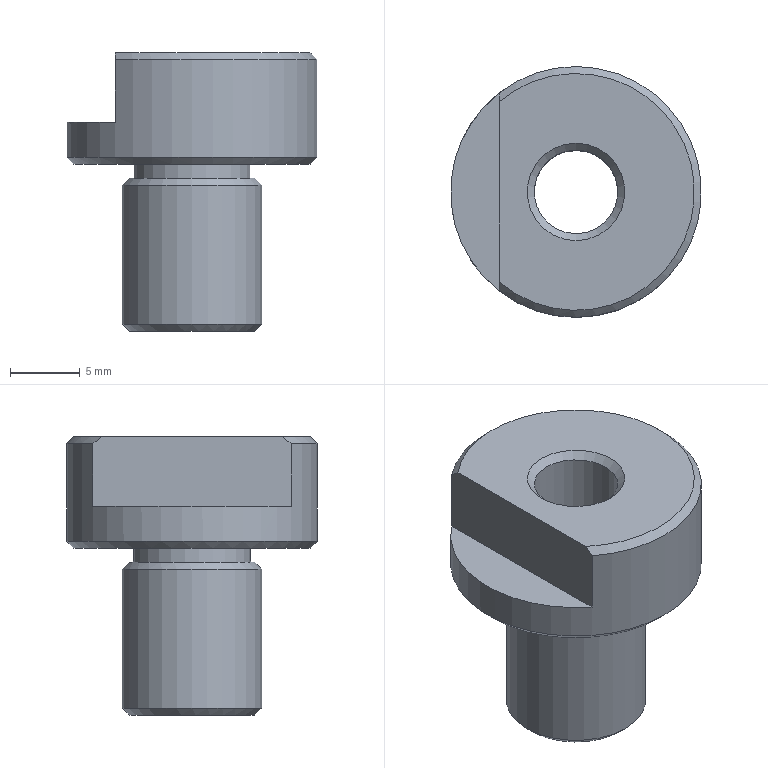Component | NX | DRILL_BUSH | 1 solid | 16 faces | box 18 x 18 x 20 mm | volume 2191 mm3 | plane 6 | cone 6 | cylinder 4 | commonest cylinder face diameters 18 x1 8.4 x1 10 x1 6 x1
STEP:
#1=CARTESIAN_POINT('',(0.,0.,0.));
#2=DIRECTION('',(0.,0.,1.));
#3=DIRECTION('',(1.,0.,0.));
#4=AXIS2_PLACEMENT_3D('',#1,#2,#3);
#5=CARTESIAN_POINT('',(12.,9.,-4.5));
#6=VERTEX_POINT('',#5);
#7=CARTESIAN_POINT('',(6.5,-7.124,-4.5));
#8=VERTEX_POINT('',#7);
#9=CARTESIAN_POINT('',(12.,0.,-4.5));
#10=DIRECTION('',(0.,0.,1.));
#11=DIRECTION('',(0.,1.,0.));
#12=AXIS2_PLACEMENT_3D('',#9,#10,#11);
#13=CIRCLE('',#12,9.);
#14=CARTESIAN_POINT('',(12.,0.,3.));
#15=DIRECTION('',(0.,0.,-1.));
#16=DIRECTION('',(0.,-1.,0.));
#17=AXIS2_PLACEMENT_3D('',#14,#15,#16);
#18=CYLINDRICAL_SURFACE('',#17,9.);
#19=CARTESIAN_POINT('',(3.142,7.5));
#20=DIRECTION('',(-1.,0.));
#21=VECTOR('',#20,1.);
#22=LINE('',#19,#21);
#23=(GEOMETRIC_REPRESENTATION_CONTEXT(2)PARAMETRIC_REPRESENTATION_CONTEXT()REPRESENTATION_CONTEXT('',''));
#24=DEFINITIONAL_REPRESENTATION('',(#22),#23);
#25=PCURVE('',#18,#24);
#26=CARTESIAN_POINT('',(12.,0.,-4.5));
#27=DIRECTION('',(0.,0.,1.));
#28=DIRECTION('',(0.,1.,0.));
#29=AXIS2_PLACEMENT_3D('',#26,#27,#28);
#30=CONICAL_SURFACE('',#29,9.,0.7854);
#31=CARTESIAN_POINT('',(0.,0.));
#32=DIRECTION('',(1.,0.));
#33=VECTOR('',#32,1.);
#34=LINE('',#31,#33);
#35=(GEOMETRIC_REPRESENTATION_CONTEXT(2)PARAMETRIC_REPRESENTATION_CONTEXT()REPRESENTATION_CONTEXT('',''));
#36=DEFINITIONAL_REPRESENTATION('',(#34),#35);
#37=PCURVE('',#30,#36);
#38=SURFACE_CURVE('',#13,(#25,#37),.PCURVE_S1.);
#39=EDGE_CURVE('',#6,#8,#38,.T.);
#40=ORIENTED_EDGE('',*,*,#39,.T.);
#41=CARTESIAN_POINT('',(6.5,-7.124,-2.));
#42=VERTEX_POINT('',#41);
#43=CARTESIAN_POINT('',(6.5,-7.124,-2.));
#44=CARTESIAN_POINT('',(6.5,-7.124,-4.5));
#45=B_SPLINE_CURVE_WITH_KNOTS('',1,(#43,#44),.UNSPECIFIED.,.F.,.F.,(2,2),(5.,7.5),.PIECEWISE_BEZIER_KNOTS.);
#46=CARTESIAN_POINT('',(0.6575,0.));
#47=DIRECTION('',(0.,1.));
#48=VECTOR('',#47,1.);
#49=LINE('',#46,#48);
#50=(GEOMETRIC_REPRESENTATION_CONTEXT(2)PARAMETRIC_REPRESENTATION_CONTEXT()REPRESENTATION_CONTEXT('',''));
#51=DEFINITIONAL_REPRESENTATION('',(#49),#50);
#52=PCURVE('',#18,#51);
#53=CARTESIAN_POINT('',(6.941,0.));
#54=DIRECTION('',(0.,1.));
#55=VECTOR('',#54,1.);
#56=LINE('',#53,#55);
#57=(GEOMETRIC_REPRESENTATION_CONTEXT(2)PARAMETRIC_REPRESENTATION_CONTEXT()REPRESENTATION_CONTEXT('',''));
#58=DEFINITIONAL_REPRESENTATION('',(#56),#57);
#59=PCURVE('',#18,#58);
#60=SEAM_CURVE('',#45,(#52,#59),.PCURVE_S1.);
#61=EDGE_CURVE('',#42,#8,#60,.T.);
#62=ORIENTED_EDGE('',*,*,#61,.F.);
#63=CARTESIAN_POINT('',(6.5,7.124,-2.));
#64=VERTEX_POINT('',#63);
#65=CARTESIAN_POINT('',(12.,0.,-2.));
#66=DIRECTION('',(0.,0.,1.));
#67=DIRECTION('',(0.,1.,0.));
#68=AXIS2_PLACEMENT_3D('',#65,#66,#67);
#69=CIRCLE('',#68,9.);
#70=CARTESIAN_POINT('',(3.142,5.));
#71=DIRECTION('',(-1.,0.));
#72=VECTOR('',#71,1.);
#73=LINE('',#70,#72);
#74=(GEOMETRIC_REPRESENTATION_CONTEXT(2)PARAMETRIC_REPRESENTATION_CONTEXT()REPRESENTATION_CONTEXT('',''));
#75=DEFINITIONAL_REPRESENTATION('',(#73),#74);
#76=PCURVE('',#18,#75);
#77=CARTESIAN_POINT('',(12.,0.,-2.));
#78=DIRECTION('',(0.,0.,1.));
#79=DIRECTION('',(0.,1.,0.));
#80=AXIS2_PLACEMENT_3D('',#77,#78,#79);
#81=PLANE('',#80);
#82=CARTESIAN_POINT('',(0.,0.));
#83=DIRECTION('',(1.,0.));
#84=AXIS2_PLACEMENT_2D('',#82,#83);
#85=CIRCLE('',#84,9.);
#86=(GEOMETRIC_REPRESENTATION_CONTEXT(2)PARAMETRIC_REPRESENTATION_CONTEXT()REPRESENTATION_CONTEXT('',''));
#87=DEFINITIONAL_REPRESENTATION('',(#85),#86);
#88=PCURVE('',#81,#87);
#89=SURFACE_CURVE('',#69,(#76,#88),.PCURVE_S1.);
#90=EDGE_CURVE('',#64,#42,#89,.T.);
#91=ORIENTED_EDGE('',*,*,#90,.F.);
#92=CARTESIAN_POINT('',(6.5,7.124,2.5));
#93=VERTEX_POINT('',#92);
#94=CARTESIAN_POINT('',(6.5,7.124,3.));
#95=DIRECTION('',(0.,0.,1.));
#96=VECTOR('',#95,1.);
#97=LINE('',#94,#96);
#98=CARTESIAN_POINT('',(2.484,0.));
#99=DIRECTION('',(0.,-1.));
#100=VECTOR('',#99,1.);
#101=LINE('',#98,#100);
#102=(GEOMETRIC_REPRESENTATION_CONTEXT(2)PARAMETRIC_REPRESENTATION_CONTEXT()REPRESENTATION_CONTEXT('',''));
#103=DEFINITIONAL_REPRESENTATION('',(#101),#102);
#104=PCURVE('',#18,#103);
#105=CARTESIAN_POINT('',(6.5,-9.7,-2.));
#106=DIRECTION('',(1.,0.,0.));
#107=DIRECTION('',(-0.,1.,0.));
#108=AXIS2_PLACEMENT_3D('',#105,#106,#107);
#109=PLANE('',#108);
#110=CARTESIAN_POINT('',(16.824,5.));
#111=DIRECTION('',(0.,1.));
#112=VECTOR('',#111,1.);
#113=LINE('',#110,#112);
#114=(GEOMETRIC_REPRESENTATION_CONTEXT(2)PARAMETRIC_REPRESENTATION_CONTEXT()REPRESENTATION_CONTEXT('',''));
#115=DEFINITIONAL_REPRESENTATION('',(#113),#114);
#116=PCURVE('',#109,#115);
#117=SURFACE_CURVE('',#97,(#104,#116),.PCURVE_S1.);
#118=EDGE_CURVE('',#64,#93,#117,.T.);
#119=ORIENTED_EDGE('',*,*,#118,.T.);
#120=CARTESIAN_POINT('',(6.5,-7.124,2.5));
#121=VERTEX_POINT('',#120);
#122=CARTESIAN_POINT('',(12.,0.,2.5));
#123=DIRECTION('',(0.,0.,-1.));
#124=DIRECTION('',(0.,1.,0.));
#125=AXIS2_PLACEMENT_3D('',#122,#123,#124);
#126=CIRCLE('',#125,9.);
#127=CARTESIAN_POINT('',(-3.142,0.5));
#128=DIRECTION('',(1.,0.));
#129=VECTOR('',#128,1.);
#130=LINE('',#127,#129);
#131=(GEOMETRIC_REPRESENTATION_CONTEXT(2)PARAMETRIC_REPRESENTATION_CONTEXT()REPRESENTATION_CONTEXT('',''));
#132=DEFINITIONAL_REPRESENTATION('',(#130),#131);
#133=PCURVE('',#18,#132);
#134=CARTESIAN_POINT('',(12.,0.,3.));
#135=DIRECTION('',(0.,0.,-1.));
#136=DIRECTION('',(0.,-1.,0.));
#137=AXIS2_PLACEMENT_3D('',#134,#135,#136);
#138=CONICAL_SURFACE('',#137,8.5,0.7854);
#139=CARTESIAN_POINT('',(-3.142,0.5));
#140=DIRECTION('',(1.,0.));
#141=VECTOR('',#140,1.);
#142=LINE('',#139,#141);
#143=(GEOMETRIC_REPRESENTATION_CONTEXT(2)PARAMETRIC_REPRESENTATION_CONTEXT()REPRESENTATION_CONTEXT('',''));
#144=DEFINITIONAL_REPRESENTATION('',(#142),#143);
#145=PCURVE('',#138,#144);
#146=SURFACE_CURVE('',#126,(#133,#145),.PCURVE_S1.);
#147=EDGE_CURVE('',#93,#121,#146,.T.);
#148=ORIENTED_EDGE('',*,*,#147,.T.);
#149=CARTESIAN_POINT('',(6.5,-7.124,3.));
#150=DIRECTION('',(0.,0.,-1.));
#151=VECTOR('',#150,1.);
#152=LINE('',#149,#151);
#153=CARTESIAN_POINT('',(6.941,0.));
#154=DIRECTION('',(0.,1.));
#155=VECTOR('',#154,1.);
#156=LINE('',#153,#155);
#157=(GEOMETRIC_REPRESENTATION_CONTEXT(2)PARAMETRIC_REPRESENTATION_CONTEXT()REPRESENTATION_CONTEXT('',''));
#158=DEFINITIONAL_REPRESENTATION('',(#156),#157);
#159=PCURVE('',#18,#158);
#160=CARTESIAN_POINT('',(2.576,5.));
#161=DIRECTION('',(0.,-1.));
#162=VECTOR('',#161,1.);
#163=LINE('',#160,#162);
#164=(GEOMETRIC_REPRESENTATION_CONTEXT(2)PARAMETRIC_REPRESENTATION_CONTEXT()REPRESENTATION_CONTEXT('',''));
#165=DEFINITIONAL_REPRESENTATION('',(#163),#164);
#166=PCURVE('',#109,#165);
#167=SURFACE_CURVE('',#152,(#159,#166),.PCURVE_S1.);
#168=EDGE_CURVE('',#121,#42,#167,.T.);
#169=ORIENTED_EDGE('',*,*,#168,.T.);
#170=ORIENTED_EDGE('',*,*,#61,.T.);
#171=CARTESIAN_POINT('',(12.,0.,-4.5));
#172=DIRECTION('',(0.,0.,1.));
#173=DIRECTION('',(0.,1.,0.));
#174=AXIS2_PLACEMENT_3D('',#171,#172,#173);
#175=CIRCLE('',#174,9.);
#176=CARTESIAN_POINT('',(9.425,7.5));
#177=DIRECTION('',(-1.,0.));
#178=VECTOR('',#177,1.);
#179=LINE('',#176,#178);
#180=(GEOMETRIC_REPRESENTATION_CONTEXT(2)PARAMETRIC_REPRESENTATION_CONTEXT()REPRESENTATION_CONTEXT('',''));
#181=DEFINITIONAL_REPRESENTATION('',(#179),#180);
#182=PCURVE('',#18,#181);
#183=CARTESIAN_POINT('',(0.,0.));
#184=DIRECTION('',(1.,0.));
#185=VECTOR('',#184,1.);
#186=LINE('',#183,#185);
#187=(GEOMETRIC_REPRESENTATION_CONTEXT(2)PARAMETRIC_REPRESENTATION_CONTEXT()REPRESENTATION_CONTEXT('',''));
#188=DEFINITIONAL_REPRESENTATION('',(#186),#187);
#189=PCURVE('',#30,#188);
#190=SURFACE_CURVE('',#175,(#182,#189),.PCURVE_S1.);
#191=EDGE_CURVE('',#8,#6,#190,.T.);
#192=ORIENTED_EDGE('',*,*,#191,.T.);
#193=EDGE_LOOP('',(#40,#62,#91,#119,#148,#169,#170,#192));
#194=FACE_BOUND('',#193,.T.);
#195=ADVANCED_FACE('',(#194),#18,.T.);
#196=CARTESIAN_POINT('',(12.,3.5,3.));
#197=VERTEX_POINT('',#196);
#198=CARTESIAN_POINT('',(12.,0.,3.));
#199=DIRECTION('',(0.,0.,-1.));
#200=DIRECTION('',(0.,1.,0.));
#201=AXIS2_PLACEMENT_3D('',#198,#199,#200);
#202=CIRCLE('',#201,3.5);
#203=CARTESIAN_POINT('',(12.,0.,3.));
#204=DIRECTION('',(0.,0.,1.));
#205=DIRECTION('',(0.,1.,0.));
#206=AXIS2_PLACEMENT_3D('',#203,#204,#205);
#207=PLANE('',#206);
#208=CARTESIAN_POINT('',(3.5,0.));
#209=CARTESIAN_POINT('',(3.5,-6.062));
#210=CARTESIAN_POINT('',(-1.75,-3.031));
#211=CARTESIAN_POINT('',(-7.,-0.));
#212=CARTESIAN_POINT('',(-1.75,3.031));
#213=CARTESIAN_POINT('',(3.5,6.062));
#214=CARTESIAN_POINT('',(3.5,0.));
#215=(BOUNDED_CURVE()B_SPLINE_CURVE(2,(#208,#209,#210,#211,#212,#213,#214),.UNSPECIFIED.,.T.,.F.)B_SPLINE_CURVE_WITH_KNOTS((1,2,2,2,2,1),(-2.094,0.,2.094,4.189,6.283,8.378),.UNSPECIFIED.)CURVE()GEOMETRIC_REPRESENTATION_ITEM()RATIONAL_B_SPLINE_CURVE((1.,0.5,1.,0.5,1.,0.5,1.))REPRESENTATION_ITEM(''));
#216=(GEOMETRIC_REPRESENTATION_CONTEXT(2)PARAMETRIC_REPRESENTATION_CONTEXT()REPRESENTATION_CONTEXT('',''));
#217=DEFINITIONAL_REPRESENTATION('',(#215),#216);
#218=PCURVE('',#207,#217);
#219=CARTESIAN_POINT('',(12.,0.,3.));
#220=DIRECTION('',(0.,0.,1.));
#221=DIRECTION('',(0.,1.,0.));
#222=AXIS2_PLACEMENT_3D('',#219,#220,#221);
#223=CONICAL_SURFACE('',#222,3.5,0.7854);
#224=CARTESIAN_POINT('',(6.283,0.));
#225=DIRECTION('',(-1.,0.));
#226=VECTOR('',#225,1.);
#227=LINE('',#224,#226);
#228=(GEOMETRIC_REPRESENTATION_CONTEXT(2)PARAMETRIC_REPRESENTATION_CONTEXT()REPRESENTATION_CONTEXT('',''));
#229=DEFINITIONAL_REPRESENTATION('',(#227),#228);
#230=PCURVE('',#223,#229);
#231=SURFACE_CURVE('',#202,(#218,#230),.PCURVE_S1.);
#232=EDGE_CURVE('',#197,#197,#231,.T.);
#233=ORIENTED_EDGE('',*,*,#232,.T.);
#234=EDGE_LOOP('',(#233));
#235=FACE_BOUND('',#234,.T.);
#236=CARTESIAN_POINT('',(6.5,-6.481,3.));
#237=VERTEX_POINT('',#236);
#238=CARTESIAN_POINT('',(6.5,6.481,3.));
#239=VERTEX_POINT('',#238);
#240=CARTESIAN_POINT('',(6.5,-9.7,3.));
#241=DIRECTION('',(-0.,1.,0.));
#242=VECTOR('',#241,1.);
#243=LINE('',#240,#242);
#244=CARTESIAN_POINT('',(-9.7,5.5));
#245=DIRECTION('',(1.,0.));
#246=VECTOR('',#245,1.);
#247=LINE('',#244,#246);
#248=(GEOMETRIC_REPRESENTATION_CONTEXT(2)PARAMETRIC_REPRESENTATION_CONTEXT()REPRESENTATION_CONTEXT('',''));
#249=DEFINITIONAL_REPRESENTATION('',(#247),#248);
#250=PCURVE('',#207,#249);
#251=CARTESIAN_POINT('',(0.,5.));
#252=DIRECTION('',(1.,0.));
#253=VECTOR('',#252,1.);
#254=LINE('',#251,#253);
#255=(GEOMETRIC_REPRESENTATION_CONTEXT(2)PARAMETRIC_REPRESENTATION_CONTEXT()REPRESENTATION_CONTEXT('',''));
#256=DEFINITIONAL_REPRESENTATION('',(#254),#255);
#257=PCURVE('',#109,#256);
#258=SURFACE_CURVE('',#243,(#250,#257),.PCURVE_S1.);
#259=EDGE_CURVE('',#237,#239,#258,.T.);
#260=ORIENTED_EDGE('',*,*,#259,.F.);
#261=CARTESIAN_POINT('',(12.,0.,3.));
#262=DIRECTION('',(0.,0.,1.));
#263=DIRECTION('',(0.,1.,0.));
#264=AXIS2_PLACEMENT_3D('',#261,#262,#263);
#265=CIRCLE('',#264,8.5);
#266=CARTESIAN_POINT('',(0.,0.));
#267=DIRECTION('',(1.,0.));
#268=AXIS2_PLACEMENT_2D('',#266,#267);
#269=CIRCLE('',#268,8.5);
#270=(GEOMETRIC_REPRESENTATION_CONTEXT(2)PARAMETRIC_REPRESENTATION_CONTEXT()REPRESENTATION_CONTEXT('',''));
#271=DEFINITIONAL_REPRESENTATION('',(#269),#270);
#272=PCURVE('',#207,#271);
#273=CARTESIAN_POINT('',(9.425,0.));
#274=DIRECTION('',(-1.,0.));
#275=VECTOR('',#274,1.);
#276=LINE('',#273,#275);
#277=(GEOMETRIC_REPRESENTATION_CONTEXT(2)PARAMETRIC_REPRESENTATION_CONTEXT()REPRESENTATION_CONTEXT('',''));
#278=DEFINITIONAL_REPRESENTATION('',(#276),#277);
#279=PCURVE('',#138,#278);
#280=SURFACE_CURVE('',#265,(#272,#279),.PCURVE_S1.);
#281=EDGE_CURVE('',#237,#239,#280,.T.);
#282=ORIENTED_EDGE('',*,*,#281,.T.);
#283=EDGE_LOOP('',(#260,#282));
#284=FACE_BOUND('',#283,.T.);
#285=ADVANCED_FACE('',(#235,#284),#207,.T.);
#286=CARTESIAN_POINT('',(12.,8.5,-5.));
#287=VERTEX_POINT('',#286);
#288=CARTESIAN_POINT('',(12.,0.,-5.));
#289=DIRECTION('',(0.,0.,-1.));
#290=DIRECTION('',(0.,1.,0.));
#291=AXIS2_PLACEMENT_3D('',#288,#289,#290);
#292=CIRCLE('',#291,8.5);
#293=CARTESIAN_POINT('',(12.,0.,-5.));
#294=DIRECTION('',(0.,0.,1.));
#295=DIRECTION('',(0.,1.,0.));
#296=AXIS2_PLACEMENT_3D('',#293,#294,#295);
#297=PLANE('',#296);
#298=CARTESIAN_POINT('',(8.5,0.));
#299=CARTESIAN_POINT('',(8.5,-14.722));
#300=CARTESIAN_POINT('',(-4.25,-7.361));
#301=CARTESIAN_POINT('',(-17.,-0.));
#302=CARTESIAN_POINT('',(-4.25,7.361));
#303=CARTESIAN_POINT('',(8.5,14.722));
#304=CARTESIAN_POINT('',(8.5,0.));
#305=(BOUNDED_CURVE()B_SPLINE_CURVE(2,(#298,#299,#300,#301,#302,#303,#304),.UNSPECIFIED.,.T.,.F.)B_SPLINE_CURVE_WITH_KNOTS((1,2,2,2,2,1),(-2.094,0.,2.094,4.189,6.283,8.378),.UNSPECIFIED.)CURVE()GEOMETRIC_REPRESENTATION_ITEM()RATIONAL_B_SPLINE_CURVE((1.,0.5,1.,0.5,1.,0.5,1.))REPRESENTATION_ITEM(''));
#306=(GEOMETRIC_REPRESENTATION_CONTEXT(2)PARAMETRIC_REPRESENTATION_CONTEXT()REPRESENTATION_CONTEXT('',''));
#307=DEFINITIONAL_REPRESENTATION('',(#305),#306);
#308=PCURVE('',#297,#307);
#309=CARTESIAN_POINT('',(6.283,-0.5));
#310=DIRECTION('',(-1.,0.));
#311=VECTOR('',#310,1.);
#312=LINE('',#309,#311);
#313=(GEOMETRIC_REPRESENTATION_CONTEXT(2)PARAMETRIC_REPRESENTATION_CONTEXT()REPRESENTATION_CONTEXT('',''));
#314=DEFINITIONAL_REPRESENTATION('',(#312),#313);
#315=PCURVE('',#30,#314);
#316=SURFACE_CURVE('',#292,(#308,#315),.PCURVE_S1.);
#317=EDGE_CURVE('',#287,#287,#316,.T.);
#318=ORIENTED_EDGE('',*,*,#317,.T.);
#319=EDGE_LOOP('',(#318));
#320=FACE_BOUND('',#319,.T.);
#321=CARTESIAN_POINT('',(12.,-4.2,-5.));
#322=VERTEX_POINT('',#321);
#323=CARTESIAN_POINT('',(12.,0.,-5.));
#324=DIRECTION('',(0.,0.,-1.));
#325=DIRECTION('',(0.,-1.,0.));
#326=AXIS2_PLACEMENT_3D('',#323,#324,#325);
#327=CIRCLE('',#326,4.2);
#328=CARTESIAN_POINT('',(-4.2,0.));
#329=CARTESIAN_POINT('',(-4.2,7.275));
#330=CARTESIAN_POINT('',(2.1,3.637));
#331=CARTESIAN_POINT('',(8.4,0.));
#332=CARTESIAN_POINT('',(2.1,-3.637));
#333=CARTESIAN_POINT('',(-4.2,-7.275));
#334=CARTESIAN_POINT('',(-4.2,0.));
#335=(BOUNDED_CURVE()B_SPLINE_CURVE(2,(#328,#329,#330,#331,#332,#333,#334),.UNSPECIFIED.,.T.,.F.)B_SPLINE_CURVE_WITH_KNOTS((1,2,2,2,2,1),(-2.094,0.,2.094,4.189,6.283,8.378),.UNSPECIFIED.)CURVE()GEOMETRIC_REPRESENTATION_ITEM()RATIONAL_B_SPLINE_CURVE((1.,0.5,1.,0.5,1.,0.5,1.))REPRESENTATION_ITEM(''));
#336=(GEOMETRIC_REPRESENTATION_CONTEXT(2)PARAMETRIC_REPRESENTATION_CONTEXT()REPRESENTATION_CONTEXT('',''));
#337=DEFINITIONAL_REPRESENTATION('',(#335),#336);
#338=PCURVE('',#297,#337);
#339=CARTESIAN_POINT('',(12.,0.,-5.5));
#340=DIRECTION('',(0.,0.,-1.));
#341=DIRECTION('',(0.,-1.,0.));
#342=AXIS2_PLACEMENT_3D('',#339,#340,#341);
#343=CYLINDRICAL_SURFACE('',#342,4.2);
#344=CARTESIAN_POINT('',(0.,-0.5));
#345=DIRECTION('',(1.,0.));
#346=VECTOR('',#345,1.);
#347=LINE('',#344,#346);
#348=(GEOMETRIC_REPRESENTATION_CONTEXT(2)PARAMETRIC_REPRESENTATION_CONTEXT()REPRESENTATION_CONTEXT('',''));
#349=DEFINITIONAL_REPRESENTATION('',(#347),#348);
#350=PCURVE('',#343,#349);
#351=SURFACE_CURVE('',#327,(#338,#350),.PCURVE_S1.);
#352=EDGE_CURVE('',#322,#322,#351,.T.);
#353=ORIENTED_EDGE('',*,*,#352,.F.);
#354=EDGE_LOOP('',(#353));
#355=FACE_BOUND('',#354,.T.);
#356=ADVANCED_FACE('',(#320,#355),#297,.F.);
#357=ORIENTED_EDGE('',*,*,#90,.T.);
#358=CARTESIAN_POINT('',(6.5,-9.7,-2.));
#359=DIRECTION('',(0.,-1.,0.));
#360=VECTOR('',#359,1.);
#361=LINE('',#358,#360);
#362=CARTESIAN_POINT('',(-9.7,5.5));
#363=DIRECTION('',(-1.,-0.));
#364=VECTOR('',#363,1.);
#365=LINE('',#362,#364);
#366=(GEOMETRIC_REPRESENTATION_CONTEXT(2)PARAMETRIC_REPRESENTATION_CONTEXT()REPRESENTATION_CONTEXT('',''));
#367=DEFINITIONAL_REPRESENTATION('',(#365),#366);
#368=PCURVE('',#81,#367);
#369=CARTESIAN_POINT('',(0.,0.));
#370=DIRECTION('',(-1.,0.));
#371=VECTOR('',#370,1.);
#372=LINE('',#369,#371);
#373=(GEOMETRIC_REPRESENTATION_CONTEXT(2)PARAMETRIC_REPRESENTATION_CONTEXT()REPRESENTATION_CONTEXT('',''));
#374=DEFINITIONAL_REPRESENTATION('',(#372),#373);
#375=PCURVE('',#109,#374);
#376=SURFACE_CURVE('',#361,(#368,#375),.PCURVE_S1.);
#377=EDGE_CURVE('',#64,#42,#376,.T.);
#378=ORIENTED_EDGE('',*,*,#377,.F.);
#379=EDGE_LOOP('',(#357,#378));
#380=FACE_BOUND('',#379,.T.);
#381=ADVANCED_FACE('',(#380),#81,.T.);
#382=ORIENTED_EDGE('',*,*,#259,.T.);
#383=CARTESIAN_POINT('',(6.5,6.481,3.));
#384=CARTESIAN_POINT('',(6.5,6.697,2.835));
#385=CARTESIAN_POINT('',(6.5,6.911,2.669));
#386=CARTESIAN_POINT('',(6.5,7.124,2.5));
#387=B_SPLINE_CURVE_WITH_KNOTS('',3,(#383,#384,#385,#386),.UNSPECIFIED.,.F.,.F.,(4,4),(0.,1.),.PIECEWISE_BEZIER_KNOTS.);
#388=CARTESIAN_POINT('',(16.181,5.));
#389=CARTESIAN_POINT('',(16.397,4.835));
#390=CARTESIAN_POINT('',(16.611,4.669));
#391=CARTESIAN_POINT('',(16.824,4.5));
#392=B_SPLINE_CURVE_WITH_KNOTS('',3,(#388,#389,#390,#391),.UNSPECIFIED.,.F.,.F.,(4,4),(0.,1.),.PIECEWISE_BEZIER_KNOTS.);
#393=(GEOMETRIC_REPRESENTATION_CONTEXT(2)PARAMETRIC_REPRESENTATION_CONTEXT()REPRESENTATION_CONTEXT('',''));
#394=DEFINITIONAL_REPRESENTATION('',(#392),#393);
#395=PCURVE('',#109,#394);
#396=CARTESIAN_POINT('',(2.438,-0.));
#397=CARTESIAN_POINT('',(2.484,0.5));
#398=B_SPLINE_CURVE_WITH_KNOTS('',1,(#396,#397),.UNSPECIFIED.,.F.,.F.,(2,2),(0.,1.),.PIECEWISE_BEZIER_KNOTS.);
#399=(GEOMETRIC_REPRESENTATION_CONTEXT(2)PARAMETRIC_REPRESENTATION_CONTEXT()REPRESENTATION_CONTEXT('',''));
#400=DEFINITIONAL_REPRESENTATION('',(#398),#399);
#401=PCURVE('',#138,#400);
#402=SURFACE_CURVE('',#387,(#395,#401),.PCURVE_S1.);
#403=EDGE_CURVE('',#239,#93,#402,.T.);
#404=ORIENTED_EDGE('',*,*,#403,.T.);
#405=ORIENTED_EDGE('',*,*,#118,.F.);
#406=ORIENTED_EDGE('',*,*,#377,.T.);
#407=ORIENTED_EDGE('',*,*,#168,.F.);
#408=CARTESIAN_POINT('',(6.5,-7.124,2.5));
#409=CARTESIAN_POINT('',(6.5,-6.911,2.669));
#410=CARTESIAN_POINT('',(6.5,-6.697,2.835));
#411=CARTESIAN_POINT('',(6.5,-6.481,3.));
#412=B_SPLINE_CURVE_WITH_KNOTS('',3,(#408,#409,#410,#411),.UNSPECIFIED.,.F.,.F.,(4,4),(0.,1.),.PIECEWISE_BEZIER_KNOTS.);
#413=CARTESIAN_POINT('',(2.576,4.5));
#414=CARTESIAN_POINT('',(2.789,4.669));
#415=CARTESIAN_POINT('',(3.003,4.835));
#416=CARTESIAN_POINT('',(3.219,5.));
#417=B_SPLINE_CURVE_WITH_KNOTS('',3,(#413,#414,#415,#416),.UNSPECIFIED.,.F.,.F.,(4,4),(0.,1.),.PIECEWISE_BEZIER_KNOTS.);
#418=(GEOMETRIC_REPRESENTATION_CONTEXT(2)PARAMETRIC_REPRESENTATION_CONTEXT()REPRESENTATION_CONTEXT('',''));
#419=DEFINITIONAL_REPRESENTATION('',(#417),#418);
#420=PCURVE('',#109,#419);
#421=CARTESIAN_POINT('',(6.941,0.5));
#422=CARTESIAN_POINT('',(6.987,-0.));
#423=B_SPLINE_CURVE_WITH_KNOTS('',1,(#421,#422),.UNSPECIFIED.,.F.,.F.,(2,2),(0.,1.),.PIECEWISE_BEZIER_KNOTS.);
#424=(GEOMETRIC_REPRESENTATION_CONTEXT(2)PARAMETRIC_REPRESENTATION_CONTEXT()REPRESENTATION_CONTEXT('',''));
#425=DEFINITIONAL_REPRESENTATION('',(#423),#424);
#426=PCURVE('',#138,#425);
#427=SURFACE_CURVE('',#412,(#420,#426),.PCURVE_S1.);
#428=EDGE_CURVE('',#121,#237,#427,.T.);
#429=ORIENTED_EDGE('',*,*,#428,.T.);
#430=EDGE_LOOP('',(#382,#404,#405,#406,#407,#429));
#431=FACE_BOUND('',#430,.T.);
#432=ADVANCED_FACE('',(#431),#109,.F.);
#433=CARTESIAN_POINT('',(12.,-4.5,-6.));
#434=VERTEX_POINT('',#433);
#435=CARTESIAN_POINT('',(12.,0.,-6.));
#436=DIRECTION('',(0.,0.,1.));
#437=DIRECTION('',(0.,-1.,0.));
#438=AXIS2_PLACEMENT_3D('',#435,#436,#437);
#439=CIRCLE('',#438,4.5);
#440=CARTESIAN_POINT('',(12.,0.,-6.));
#441=DIRECTION('',(0.,0.,-1.));
#442=DIRECTION('',(0.,-1.,0.));
#443=AXIS2_PLACEMENT_3D('',#440,#441,#442);
#444=PLANE('',#443);
#445=CARTESIAN_POINT('',(4.5,0.));
#446=CARTESIAN_POINT('',(4.5,-7.794));
#447=CARTESIAN_POINT('',(-2.25,-3.897));
#448=CARTESIAN_POINT('',(-9.,-0.));
#449=CARTESIAN_POINT('',(-2.25,3.897));
#450=CARTESIAN_POINT('',(4.5,7.794));
#451=CARTESIAN_POINT('',(4.5,0.));
#452=(BOUNDED_CURVE()B_SPLINE_CURVE(2,(#445,#446,#447,#448,#449,#450,#451),.UNSPECIFIED.,.T.,.F.)B_SPLINE_CURVE_WITH_KNOTS((1,2,2,2,2,1),(-2.094,0.,2.094,4.189,6.283,8.378),.UNSPECIFIED.)CURVE()GEOMETRIC_REPRESENTATION_ITEM()RATIONAL_B_SPLINE_CURVE((1.,0.5,1.,0.5,1.,0.5,1.))REPRESENTATION_ITEM(''));
#453=(GEOMETRIC_REPRESENTATION_CONTEXT(2)PARAMETRIC_REPRESENTATION_CONTEXT()REPRESENTATION_CONTEXT('',''));
#454=DEFINITIONAL_REPRESENTATION('',(#452),#453);
#455=PCURVE('',#444,#454);
#456=CARTESIAN_POINT('',(12.,0.,-6.5));
#457=DIRECTION('',(0.,0.,-1.));
#458=DIRECTION('',(0.,-1.,0.));
#459=AXIS2_PLACEMENT_3D('',#456,#457,#458);
#460=CONICAL_SURFACE('',#459,5.,0.7854);
#461=CARTESIAN_POINT('',(6.283,-0.5));
#462=DIRECTION('',(-1.,0.));
#463=VECTOR('',#462,1.);
#464=LINE('',#461,#463);
#465=(GEOMETRIC_REPRESENTATION_CONTEXT(2)PARAMETRIC_REPRESENTATION_CONTEXT()REPRESENTATION_CONTEXT('',''));
#466=DEFINITIONAL_REPRESENTATION('',(#464),#465);
#467=PCURVE('',#460,#466);
#468=SURFACE_CURVE('',#439,(#455,#467),.PCURVE_S1.);
#469=EDGE_CURVE('',#434,#434,#468,.T.);
#470=ORIENTED_EDGE('',*,*,#469,.T.);
#471=EDGE_LOOP('',(#470));
#472=FACE_BOUND('',#471,.T.);
#473=CARTESIAN_POINT('',(12.,-4.2,-6.));
#474=VERTEX_POINT('',#473);
#475=CARTESIAN_POINT('',(12.,0.,-6.));
#476=DIRECTION('',(0.,0.,1.));
#477=DIRECTION('',(0.,-1.,0.));
#478=AXIS2_PLACEMENT_3D('',#475,#476,#477);
#479=CIRCLE('',#478,4.2);
#480=CARTESIAN_POINT('',(4.2,0.));
#481=CARTESIAN_POINT('',(4.2,-7.275));
#482=CARTESIAN_POINT('',(-2.1,-3.637));
#483=CARTESIAN_POINT('',(-8.4,-0.));
#484=CARTESIAN_POINT('',(-2.1,3.637));
#485=CARTESIAN_POINT('',(4.2,7.275));
#486=CARTESIAN_POINT('',(4.2,0.));
#487=(BOUNDED_CURVE()B_SPLINE_CURVE(2,(#480,#481,#482,#483,#484,#485,#486),.UNSPECIFIED.,.T.,.F.)B_SPLINE_CURVE_WITH_KNOTS((1,2,2,2,2,1),(-2.094,0.,2.094,4.189,6.283,8.378),.UNSPECIFIED.)CURVE()GEOMETRIC_REPRESENTATION_ITEM()RATIONAL_B_SPLINE_CURVE((1.,0.5,1.,0.5,1.,0.5,1.))REPRESENTATION_ITEM(''));
#488=(GEOMETRIC_REPRESENTATION_CONTEXT(2)PARAMETRIC_REPRESENTATION_CONTEXT()REPRESENTATION_CONTEXT('',''));
#489=DEFINITIONAL_REPRESENTATION('',(#487),#488);
#490=PCURVE('',#444,#489);
#491=CARTESIAN_POINT('',(6.283,0.5));
#492=DIRECTION('',(-1.,0.));
#493=VECTOR('',#492,1.);
#494=LINE('',#491,#493);
#495=(GEOMETRIC_REPRESENTATION_CONTEXT(2)PARAMETRIC_REPRESENTATION_CONTEXT()REPRESENTATION_CONTEXT('',''));
#496=DEFINITIONAL_REPRESENTATION('',(#494),#495);
#497=PCURVE('',#343,#496);
#498=SURFACE_CURVE('',#479,(#490,#497),.PCURVE_S1.);
#499=EDGE_CURVE('',#474,#474,#498,.T.);
#500=ORIENTED_EDGE('',*,*,#499,.F.);
#501=EDGE_LOOP('',(#500));
#502=FACE_BOUND('',#501,.T.);
#503=ADVANCED_FACE('',(#472,#502),#444,.F.);
#504=ORIENTED_EDGE('',*,*,#499,.T.);
#505=CARTESIAN_POINT('',(12.,-4.2,-5.));
#506=CARTESIAN_POINT('',(12.,-4.2,-6.));
#507=B_SPLINE_CURVE_WITH_KNOTS('',1,(#505,#506),.UNSPECIFIED.,.F.,.F.,(2,2),(-0.5,0.5),.PIECEWISE_BEZIER_KNOTS.);
#508=CARTESIAN_POINT('',(0.,0.));
#509=DIRECTION('',(0.,1.));
#510=VECTOR('',#509,1.);
#511=LINE('',#508,#510);
#512=(GEOMETRIC_REPRESENTATION_CONTEXT(2)PARAMETRIC_REPRESENTATION_CONTEXT()REPRESENTATION_CONTEXT('',''));
#513=DEFINITIONAL_REPRESENTATION('',(#511),#512);
#514=PCURVE('',#343,#513);
#515=CARTESIAN_POINT('',(6.283,0.));
#516=DIRECTION('',(0.,1.));
#517=VECTOR('',#516,1.);
#518=LINE('',#515,#517);
#519=(GEOMETRIC_REPRESENTATION_CONTEXT(2)PARAMETRIC_REPRESENTATION_CONTEXT()REPRESENTATION_CONTEXT('',''));
#520=DEFINITIONAL_REPRESENTATION('',(#518),#519);
#521=PCURVE('',#343,#520);
#522=SEAM_CURVE('',#507,(#514,#521),.PCURVE_S1.);
#523=EDGE_CURVE('',#322,#474,#522,.T.);
#524=ORIENTED_EDGE('',*,*,#523,.F.);
#525=ORIENTED_EDGE('',*,*,#352,.T.);
#526=ORIENTED_EDGE('',*,*,#523,.T.);
#527=EDGE_LOOP('',(#504,#524,#525,#526));
#528=FACE_BOUND('',#527,.T.);
#529=ADVANCED_FACE('',(#528),#343,.T.);
#530=CARTESIAN_POINT('',(12.,3.5,-17.));
#531=VERTEX_POINT('',#530);
#532=CARTESIAN_POINT('',(12.,0.,-17.));
#533=DIRECTION('',(0.,0.,1.));
#534=DIRECTION('',(0.,1.,0.));
#535=AXIS2_PLACEMENT_3D('',#532,#533,#534);
#536=CIRCLE('',#535,3.5);
#537=CARTESIAN_POINT('',(12.,0.,-17.));
#538=DIRECTION('',(0.,0.,1.));
#539=DIRECTION('',(0.,1.,0.));
#540=AXIS2_PLACEMENT_3D('',#537,#538,#539);
#541=PLANE('',#540);
#542=CARTESIAN_POINT('',(0.,0.));
#543=DIRECTION('',(1.,0.));
#544=AXIS2_PLACEMENT_2D('',#542,#543);
#545=CIRCLE('',#544,3.5);
#546=(GEOMETRIC_REPRESENTATION_CONTEXT(2)PARAMETRIC_REPRESENTATION_CONTEXT()REPRESENTATION_CONTEXT('',''));
#547=DEFINITIONAL_REPRESENTATION('',(#545),#546);
#548=PCURVE('',#541,#547);
#549=CARTESIAN_POINT('',(12.,0.,-17.));
#550=DIRECTION('',(0.,0.,-1.));
#551=DIRECTION('',(0.,-1.,0.));
#552=AXIS2_PLACEMENT_3D('',#549,#550,#551);
#553=CONICAL_SURFACE('',#552,3.5,0.7854);
#554=CARTESIAN_POINT('',(9.425,0.));
#555=DIRECTION('',(-1.,0.));
#556=VECTOR('',#555,1.);
#557=LINE('',#554,#556);
#558=(GEOMETRIC_REPRESENTATION_CONTEXT(2)PARAMETRIC_REPRESENTATION_CONTEXT()REPRESENTATION_CONTEXT('',''));
#559=DEFINITIONAL_REPRESENTATION('',(#557),#558);
#560=PCURVE('',#553,#559);
#561=SURFACE_CURVE('',#536,(#548,#560),.PCURVE_S1.);
#562=EDGE_CURVE('',#531,#531,#561,.T.);
#563=ORIENTED_EDGE('',*,*,#562,.T.);
#564=EDGE_LOOP('',(#563));
#565=FACE_BOUND('',#564,.T.);
#566=CARTESIAN_POINT('',(12.,4.5,-17.));
#567=VERTEX_POINT('',#566);
#568=CARTESIAN_POINT('',(12.,0.,-17.));
#569=DIRECTION('',(0.,0.,-1.));
#570=DIRECTION('',(0.,1.,0.));
#571=AXIS2_PLACEMENT_3D('',#568,#569,#570);
#572=CIRCLE('',#571,4.5);
#573=CARTESIAN_POINT('',(4.5,0.));
#574=CARTESIAN_POINT('',(4.5,-7.794));
#575=CARTESIAN_POINT('',(-2.25,-3.897));
#576=CARTESIAN_POINT('',(-9.,-0.));
#577=CARTESIAN_POINT('',(-2.25,3.897));
#578=CARTESIAN_POINT('',(4.5,7.794));
#579=CARTESIAN_POINT('',(4.5,0.));
#580=(BOUNDED_CURVE()B_SPLINE_CURVE(2,(#573,#574,#575,#576,#577,#578,#579),.UNSPECIFIED.,.T.,.F.)B_SPLINE_CURVE_WITH_KNOTS((1,2,2,2,2,1),(-2.094,0.,2.094,4.189,6.283,8.378),.UNSPECIFIED.)CURVE()GEOMETRIC_REPRESENTATION_ITEM()RATIONAL_B_SPLINE_CURVE((1.,0.5,1.,0.5,1.,0.5,1.))REPRESENTATION_ITEM(''));
#581=(GEOMETRIC_REPRESENTATION_CONTEXT(2)PARAMETRIC_REPRESENTATION_CONTEXT()REPRESENTATION_CONTEXT('',''));
#582=DEFINITIONAL_REPRESENTATION('',(#580),#581);
#583=PCURVE('',#541,#582);
#584=CARTESIAN_POINT('',(12.,0.,-16.5));
#585=DIRECTION('',(0.,0.,1.));
#586=DIRECTION('',(0.,1.,0.));
#587=AXIS2_PLACEMENT_3D('',#584,#585,#586);
#588=CONICAL_SURFACE('',#587,5.,0.7854);
#589=CARTESIAN_POINT('',(6.283,-0.5));
#590=DIRECTION('',(-1.,0.));
#591=VECTOR('',#590,1.);
#592=LINE('',#589,#591);
#593=(GEOMETRIC_REPRESENTATION_CONTEXT(2)PARAMETRIC_REPRESENTATION_CONTEXT()REPRESENTATION_CONTEXT('',''));
#594=DEFINITIONAL_REPRESENTATION('',(#592),#593);
#595=PCURVE('',#588,#594);
#596=SURFACE_CURVE('',#572,(#583,#595),.PCURVE_S1.);
#597=EDGE_CURVE('',#567,#567,#596,.T.);
#598=ORIENTED_EDGE('',*,*,#597,.T.);
#599=EDGE_LOOP('',(#598));
#600=FACE_BOUND('',#599,.T.);
#601=ADVANCED_FACE('',(#565,#600),#541,.F.);
#602=CARTESIAN_POINT('',(12.,5.,-16.5));
#603=VERTEX_POINT('',#602);
#604=CARTESIAN_POINT('',(12.,-5.,-16.5));
#605=VERTEX_POINT('',#604);
#606=CARTESIAN_POINT('',(12.,0.,-16.5));
#607=DIRECTION('',(0.,0.,1.));
#608=DIRECTION('',(0.,1.,0.));
#609=AXIS2_PLACEMENT_3D('',#606,#607,#608);
#610=CIRCLE('',#609,5.);
#611=CARTESIAN_POINT('',(12.,0.,-5.));
#612=DIRECTION('',(0.,0.,-1.));
#613=DIRECTION('',(0.,-1.,0.));
#614=AXIS2_PLACEMENT_3D('',#611,#612,#613);
#615=CYLINDRICAL_SURFACE('',#614,5.);
#616=CARTESIAN_POINT('',(3.142,11.5));
#617=DIRECTION('',(-1.,0.));
#618=VECTOR('',#617,1.);
#619=LINE('',#616,#618);
#620=(GEOMETRIC_REPRESENTATION_CONTEXT(2)PARAMETRIC_REPRESENTATION_CONTEXT()REPRESENTATION_CONTEXT('',''));
#621=DEFINITIONAL_REPRESENTATION('',(#619),#620);
#622=PCURVE('',#615,#621);
#623=CARTESIAN_POINT('',(0.,0.));
#624=DIRECTION('',(1.,0.));
#625=VECTOR('',#624,1.);
#626=LINE('',#623,#625);
#627=(GEOMETRIC_REPRESENTATION_CONTEXT(2)PARAMETRIC_REPRESENTATION_CONTEXT()REPRESENTATION_CONTEXT('',''));
#628=DEFINITIONAL_REPRESENTATION('',(#626),#627);
#629=PCURVE('',#588,#628);
#630=SURFACE_CURVE('',#610,(#622,#629),.PCURVE_S1.);
#631=EDGE_CURVE('',#603,#605,#630,.T.);
#632=ORIENTED_EDGE('',*,*,#631,.T.);
#633=CARTESIAN_POINT('',(12.,-5.,-6.5));
#634=VERTEX_POINT('',#633);
#635=CARTESIAN_POINT('',(12.,-5.,-6.5));
#636=CARTESIAN_POINT('',(12.,-5.,-16.5));
#637=B_SPLINE_CURVE_WITH_KNOTS('',1,(#635,#636),.UNSPECIFIED.,.F.,.F.,(2,2),(1.5,11.5),.PIECEWISE_BEZIER_KNOTS.);
#638=CARTESIAN_POINT('',(0.,0.));
#639=DIRECTION('',(0.,1.));
#640=VECTOR('',#639,1.);
#641=LINE('',#638,#640);
#642=(GEOMETRIC_REPRESENTATION_CONTEXT(2)PARAMETRIC_REPRESENTATION_CONTEXT()REPRESENTATION_CONTEXT('',''));
#643=DEFINITIONAL_REPRESENTATION('',(#641),#642);
#644=PCURVE('',#615,#643);
#645=CARTESIAN_POINT('',(6.283,0.));
#646=DIRECTION('',(0.,1.));
#647=VECTOR('',#646,1.);
#648=LINE('',#645,#647);
#649=(GEOMETRIC_REPRESENTATION_CONTEXT(2)PARAMETRIC_REPRESENTATION_CONTEXT()REPRESENTATION_CONTEXT('',''));
#650=DEFINITIONAL_REPRESENTATION('',(#648),#649);
#651=PCURVE('',#615,#650);
#652=SEAM_CURVE('',#637,(#644,#651),.PCURVE_S1.);
#653=EDGE_CURVE('',#634,#605,#652,.T.);
#654=ORIENTED_EDGE('',*,*,#653,.F.);
#655=CARTESIAN_POINT('',(12.,0.,-6.5));
#656=DIRECTION('',(0.,0.,-1.));
#657=DIRECTION('',(0.,-1.,0.));
#658=AXIS2_PLACEMENT_3D('',#655,#656,#657);
#659=CIRCLE('',#658,5.);
#660=CARTESIAN_POINT('',(0.,1.5));
#661=DIRECTION('',(1.,0.));
#662=VECTOR('',#661,1.);
#663=LINE('',#660,#662);
#664=(GEOMETRIC_REPRESENTATION_CONTEXT(2)PARAMETRIC_REPRESENTATION_CONTEXT()REPRESENTATION_CONTEXT('',''));
#665=DEFINITIONAL_REPRESENTATION('',(#663),#664);
#666=PCURVE('',#615,#665);
#667=CARTESIAN_POINT('',(0.,0.));
#668=DIRECTION('',(1.,0.));
#669=VECTOR('',#668,1.);
#670=LINE('',#667,#669);
#671=(GEOMETRIC_REPRESENTATION_CONTEXT(2)PARAMETRIC_REPRESENTATION_CONTEXT()REPRESENTATION_CONTEXT('',''));
#672=DEFINITIONAL_REPRESENTATION('',(#670),#671);
#673=PCURVE('',#460,#672);
#674=SURFACE_CURVE('',#659,(#666,#673),.PCURVE_S1.);
#675=EDGE_CURVE('',#634,#634,#674,.T.);
#676=ORIENTED_EDGE('',*,*,#675,.T.);
#677=ORIENTED_EDGE('',*,*,#653,.T.);
#678=CARTESIAN_POINT('',(12.,0.,-16.5));
#679=DIRECTION('',(0.,0.,1.));
#680=DIRECTION('',(0.,1.,0.));
#681=AXIS2_PLACEMENT_3D('',#678,#679,#680);
#682=CIRCLE('',#681,5.);
#683=CARTESIAN_POINT('',(9.425,11.5));
#684=DIRECTION('',(-1.,0.));
#685=VECTOR('',#684,1.);
#686=LINE('',#683,#685);
#687=(GEOMETRIC_REPRESENTATION_CONTEXT(2)PARAMETRIC_REPRESENTATION_CONTEXT()REPRESENTATION_CONTEXT('',''));
#688=DEFINITIONAL_REPRESENTATION('',(#686),#687);
#689=PCURVE('',#615,#688);
#690=CARTESIAN_POINT('',(0.,0.));
#691=DIRECTION('',(1.,0.));
#692=VECTOR('',#691,1.);
#693=LINE('',#690,#692);
#694=(GEOMETRIC_REPRESENTATION_CONTEXT(2)PARAMETRIC_REPRESENTATION_CONTEXT()REPRESENTATION_CONTEXT('',''));
#695=DEFINITIONAL_REPRESENTATION('',(#693),#694);
#696=PCURVE('',#588,#695);
#697=SURFACE_CURVE('',#682,(#689,#696),.PCURVE_S1.);
#698=EDGE_CURVE('',#605,#603,#697,.T.);
#699=ORIENTED_EDGE('',*,*,#698,.T.);
#700=EDGE_LOOP('',(#632,#654,#676,#677,#699));
#701=FACE_BOUND('',#700,.T.);
#702=ADVANCED_FACE('',(#701),#615,.T.);
#703=CARTESIAN_POINT('',(12.,3.,-16.5));
#704=VERTEX_POINT('',#703);
#705=CARTESIAN_POINT('',(12.,0.,-16.5));
#706=DIRECTION('',(0.,0.,-1.));
#707=DIRECTION('',(0.,1.,0.));
#708=AXIS2_PLACEMENT_3D('',#705,#706,#707);
#709=CIRCLE('',#708,3.);
#710=CARTESIAN_POINT('',(12.,0.,3.));
#711=DIRECTION('',(0.,0.,-1.));
#712=DIRECTION('',(0.,-1.,0.));
#713=AXIS2_PLACEMENT_3D('',#710,#711,#712);
#714=CYLINDRICAL_SURFACE('',#713,3.);
#715=CARTESIAN_POINT('',(3.142,19.5));
#716=DIRECTION('',(1.,0.));
#717=VECTOR('',#716,1.);
#718=LINE('',#715,#717);
#719=(GEOMETRIC_REPRESENTATION_CONTEXT(2)PARAMETRIC_REPRESENTATION_CONTEXT()REPRESENTATION_CONTEXT('',''));
#720=DEFINITIONAL_REPRESENTATION('',(#718),#719);
#721=PCURVE('',#714,#720);
#722=CARTESIAN_POINT('',(3.142,-0.5));
#723=DIRECTION('',(1.,0.));
#724=VECTOR('',#723,1.);
#725=LINE('',#722,#724);
#726=(GEOMETRIC_REPRESENTATION_CONTEXT(2)PARAMETRIC_REPRESENTATION_CONTEXT()REPRESENTATION_CONTEXT('',''));
#727=DEFINITIONAL_REPRESENTATION('',(#725),#726);
#728=PCURVE('',#553,#727);
#729=SURFACE_CURVE('',#709,(#721,#728),.PCURVE_S1.);
#730=EDGE_CURVE('',#704,#704,#729,.T.);
#731=ORIENTED_EDGE('',*,*,#730,.F.);
#732=CARTESIAN_POINT('',(12.,3.,2.5));
#733=VERTEX_POINT('',#732);
#734=CARTESIAN_POINT('',(12.,3.,2.5));
#735=CARTESIAN_POINT('',(12.,3.,-16.5));
#736=B_SPLINE_CURVE_WITH_KNOTS('',1,(#734,#735),.UNSPECIFIED.,.F.,.F.,(2,2),(0.5,19.5),.PIECEWISE_BEZIER_KNOTS.);
#737=CARTESIAN_POINT('',(3.142,0.));
#738=DIRECTION('',(0.,1.));
#739=VECTOR('',#738,1.);
#740=LINE('',#737,#739);
#741=(GEOMETRIC_REPRESENTATION_CONTEXT(2)PARAMETRIC_REPRESENTATION_CONTEXT()REPRESENTATION_CONTEXT('',''));
#742=DEFINITIONAL_REPRESENTATION('',(#740),#741);
#743=PCURVE('',#714,#742);
#744=CARTESIAN_POINT('',(9.425,0.));
#745=DIRECTION('',(0.,1.));
#746=VECTOR('',#745,1.);
#747=LINE('',#744,#746);
#748=(GEOMETRIC_REPRESENTATION_CONTEXT(2)PARAMETRIC_REPRESENTATION_CONTEXT()REPRESENTATION_CONTEXT('',''));
#749=DEFINITIONAL_REPRESENTATION('',(#747),#748);
#750=PCURVE('',#714,#749);
#751=SEAM_CURVE('',#736,(#743,#750),.PCURVE_S1.);
#752=EDGE_CURVE('',#733,#704,#751,.T.);
#753=ORIENTED_EDGE('',*,*,#752,.F.);
#754=CARTESIAN_POINT('',(12.,0.,2.5));
#755=DIRECTION('',(0.,0.,1.));
#756=DIRECTION('',(0.,1.,0.));
#757=AXIS2_PLACEMENT_3D('',#754,#755,#756);
#758=CIRCLE('',#757,3.);
#759=CARTESIAN_POINT('',(9.425,0.5));
#760=DIRECTION('',(-1.,0.));
#761=VECTOR('',#760,1.);
#762=LINE('',#759,#761);
#763=(GEOMETRIC_REPRESENTATION_CONTEXT(2)PARAMETRIC_REPRESENTATION_CONTEXT()REPRESENTATION_CONTEXT('',''));
#764=DEFINITIONAL_REPRESENTATION('',(#762),#763);
#765=PCURVE('',#714,#764);
#766=CARTESIAN_POINT('',(0.,-0.5));
#767=DIRECTION('',(1.,0.));
#768=VECTOR('',#767,1.);
#769=LINE('',#766,#768);
#770=(GEOMETRIC_REPRESENTATION_CONTEXT(2)PARAMETRIC_REPRESENTATION_CONTEXT()REPRESENTATION_CONTEXT('',''));
#771=DEFINITIONAL_REPRESENTATION('',(#769),#770);
#772=PCURVE('',#223,#771);
#773=SURFACE_CURVE('',#758,(#765,#772),.PCURVE_S1.);
#774=EDGE_CURVE('',#733,#733,#773,.T.);
#775=ORIENTED_EDGE('',*,*,#774,.F.);
#776=ORIENTED_EDGE('',*,*,#752,.T.);
#777=EDGE_LOOP('',(#731,#753,#775,#776));
#778=FACE_BOUND('',#777,.F.);
#779=ADVANCED_FACE('',(#778),#714,.F.);
#780=ORIENTED_EDGE('',*,*,#730,.T.);
#781=CARTESIAN_POINT('',(12.,3.,-16.5));
#782=CARTESIAN_POINT('',(12.,3.5,-17.));
#783=B_SPLINE_CURVE_WITH_KNOTS('',1,(#781,#782),.UNSPECIFIED.,.F.,.F.,(2,2),(-0.7071,0.),.PIECEWISE_BEZIER_KNOTS.);
#784=CARTESIAN_POINT('',(9.425,0.));
#785=DIRECTION('',(0.,1.));
#786=VECTOR('',#785,1.);
#787=LINE('',#784,#786);
#788=(GEOMETRIC_REPRESENTATION_CONTEXT(2)PARAMETRIC_REPRESENTATION_CONTEXT()REPRESENTATION_CONTEXT('',''));
#789=DEFINITIONAL_REPRESENTATION('',(#787),#788);
#790=PCURVE('',#553,#789);
#791=CARTESIAN_POINT('',(3.142,0.));
#792=DIRECTION('',(0.,1.));
#793=VECTOR('',#792,1.);
#794=LINE('',#791,#793);
#795=(GEOMETRIC_REPRESENTATION_CONTEXT(2)PARAMETRIC_REPRESENTATION_CONTEXT()REPRESENTATION_CONTEXT('',''));
#796=DEFINITIONAL_REPRESENTATION('',(#794),#795);
#797=PCURVE('',#553,#796);
#798=SEAM_CURVE('',#783,(#790,#797),.PCURVE_S1.);
#799=EDGE_CURVE('',#704,#531,#798,.T.);
#800=ORIENTED_EDGE('',*,*,#799,.T.);
#801=ORIENTED_EDGE('',*,*,#562,.T.);
#802=ORIENTED_EDGE('',*,*,#799,.F.);
#803=EDGE_LOOP('',(#780,#800,#801,#802));
#804=FACE_BOUND('',#803,.F.);
#805=ADVANCED_FACE('',(#804),#553,.F.);
#806=ORIENTED_EDGE('',*,*,#597,.F.);
#807=CARTESIAN_POINT('',(12.,4.5,-17.));
#808=CARTESIAN_POINT('',(12.,5.,-16.5));
#809=B_SPLINE_CURVE_WITH_KNOTS('',1,(#807,#808),.UNSPECIFIED.,.F.,.F.,(2,2),(-0.7071,0.),.PIECEWISE_BEZIER_KNOTS.);
#810=CARTESIAN_POINT('',(6.283,0.));
#811=DIRECTION('',(0.,1.));
#812=VECTOR('',#811,1.);
#813=LINE('',#810,#812);
#814=(GEOMETRIC_REPRESENTATION_CONTEXT(2)PARAMETRIC_REPRESENTATION_CONTEXT()REPRESENTATION_CONTEXT('',''));
#815=DEFINITIONAL_REPRESENTATION('',(#813),#814);
#816=PCURVE('',#588,#815);
#817=CARTESIAN_POINT('',(0.,0.));
#818=DIRECTION('',(0.,1.));
#819=VECTOR('',#818,1.);
#820=LINE('',#817,#819);
#821=(GEOMETRIC_REPRESENTATION_CONTEXT(2)PARAMETRIC_REPRESENTATION_CONTEXT()REPRESENTATION_CONTEXT('',''));
#822=DEFINITIONAL_REPRESENTATION('',(#820),#821);
#823=PCURVE('',#588,#822);
#824=SEAM_CURVE('',#809,(#816,#823),.PCURVE_S1.);
#825=EDGE_CURVE('',#567,#603,#824,.T.);
#826=ORIENTED_EDGE('',*,*,#825,.T.);
#827=ORIENTED_EDGE('',*,*,#698,.F.);
#828=ORIENTED_EDGE('',*,*,#631,.F.);
#829=ORIENTED_EDGE('',*,*,#825,.F.);
#830=EDGE_LOOP('',(#806,#826,#827,#828,#829));
#831=FACE_BOUND('',#830,.T.);
#832=ADVANCED_FACE('',(#831),#588,.T.);
#833=ORIENTED_EDGE('',*,*,#469,.F.);
#834=CARTESIAN_POINT('',(12.,-4.5,-6.));
#835=CARTESIAN_POINT('',(12.,-5.,-6.5));
#836=B_SPLINE_CURVE_WITH_KNOTS('',1,(#834,#835),.UNSPECIFIED.,.F.,.F.,(2,2),(-0.7071,0.),.PIECEWISE_BEZIER_KNOTS.);
#837=CARTESIAN_POINT('',(6.283,0.));
#838=DIRECTION('',(0.,1.));
#839=VECTOR('',#838,1.);
#840=LINE('',#837,#839);
#841=(GEOMETRIC_REPRESENTATION_CONTEXT(2)PARAMETRIC_REPRESENTATION_CONTEXT()REPRESENTATION_CONTEXT('',''));
#842=DEFINITIONAL_REPRESENTATION('',(#840),#841);
#843=PCURVE('',#460,#842);
#844=CARTESIAN_POINT('',(0.,0.));
#845=DIRECTION('',(0.,1.));
#846=VECTOR('',#845,1.);
#847=LINE('',#844,#846);
#848=(GEOMETRIC_REPRESENTATION_CONTEXT(2)PARAMETRIC_REPRESENTATION_CONTEXT()REPRESENTATION_CONTEXT('',''));
#849=DEFINITIONAL_REPRESENTATION('',(#847),#848);
#850=PCURVE('',#460,#849);
#851=SEAM_CURVE('',#836,(#843,#850),.PCURVE_S1.);
#852=EDGE_CURVE('',#434,#634,#851,.T.);
#853=ORIENTED_EDGE('',*,*,#852,.T.);
#854=ORIENTED_EDGE('',*,*,#675,.F.);
#855=ORIENTED_EDGE('',*,*,#852,.F.);
#856=EDGE_LOOP('',(#833,#853,#854,#855));
#857=FACE_BOUND('',#856,.T.);
#858=ADVANCED_FACE('',(#857),#460,.T.);
#859=ORIENTED_EDGE('',*,*,#317,.F.);
#860=CARTESIAN_POINT('',(12.,8.5,-5.));
#861=CARTESIAN_POINT('',(12.,9.,-4.5));
#862=B_SPLINE_CURVE_WITH_KNOTS('',1,(#860,#861),.UNSPECIFIED.,.F.,.F.,(2,2),(-0.7071,0.),.PIECEWISE_BEZIER_KNOTS.);
#863=CARTESIAN_POINT('',(6.283,0.));
#864=DIRECTION('',(0.,1.));
#865=VECTOR('',#864,1.);
#866=LINE('',#863,#865);
#867=(GEOMETRIC_REPRESENTATION_CONTEXT(2)PARAMETRIC_REPRESENTATION_CONTEXT()REPRESENTATION_CONTEXT('',''));
#868=DEFINITIONAL_REPRESENTATION('',(#866),#867);
#869=PCURVE('',#30,#868);
#870=CARTESIAN_POINT('',(0.,0.));
#871=DIRECTION('',(0.,1.));
#872=VECTOR('',#871,1.);
#873=LINE('',#870,#872);
#874=(GEOMETRIC_REPRESENTATION_CONTEXT(2)PARAMETRIC_REPRESENTATION_CONTEXT()REPRESENTATION_CONTEXT('',''));
#875=DEFINITIONAL_REPRESENTATION('',(#873),#874);
#876=PCURVE('',#30,#875);
#877=SEAM_CURVE('',#862,(#869,#876),.PCURVE_S1.);
#878=EDGE_CURVE('',#287,#6,#877,.T.);
#879=ORIENTED_EDGE('',*,*,#878,.T.);
#880=ORIENTED_EDGE('',*,*,#191,.F.);
#881=ORIENTED_EDGE('',*,*,#39,.F.);
#882=ORIENTED_EDGE('',*,*,#878,.F.);
#883=EDGE_LOOP('',(#859,#879,#880,#881,#882));
#884=FACE_BOUND('',#883,.T.);
#885=ADVANCED_FACE('',(#884),#30,.T.);
#886=ORIENTED_EDGE('',*,*,#428,.F.);
#887=ORIENTED_EDGE('',*,*,#147,.F.);
#888=ORIENTED_EDGE('',*,*,#403,.F.);
#889=ORIENTED_EDGE('',*,*,#281,.F.);
#890=EDGE_LOOP('',(#886,#887,#888,#889));
#891=FACE_BOUND('',#890,.T.);
#892=ADVANCED_FACE('',(#891),#138,.T.);
#893=ORIENTED_EDGE('',*,*,#774,.T.);
#894=CARTESIAN_POINT('',(12.,3.,2.5));
#895=CARTESIAN_POINT('',(12.,3.5,3.));
#896=B_SPLINE_CURVE_WITH_KNOTS('',1,(#894,#895),.UNSPECIFIED.,.F.,.F.,(2,2),(-0.7071,0.),.PIECEWISE_BEZIER_KNOTS.);
#897=CARTESIAN_POINT('',(6.283,0.));
#898=DIRECTION('',(0.,1.));
#899=VECTOR('',#898,1.);
#900=LINE('',#897,#899);
#901=(GEOMETRIC_REPRESENTATION_CONTEXT(2)PARAMETRIC_REPRESENTATION_CONTEXT()REPRESENTATION_CONTEXT('',''));
#902=DEFINITIONAL_REPRESENTATION('',(#900),#901);
#903=PCURVE('',#223,#902);
#904=CARTESIAN_POINT('',(0.,0.));
#905=DIRECTION('',(0.,1.));
#906=VECTOR('',#905,1.);
#907=LINE('',#904,#906);
#908=(GEOMETRIC_REPRESENTATION_CONTEXT(2)PARAMETRIC_REPRESENTATION_CONTEXT()REPRESENTATION_CONTEXT('',''));
#909=DEFINITIONAL_REPRESENTATION('',(#907),#908);
#910=PCURVE('',#223,#909);
#911=SEAM_CURVE('',#896,(#903,#910),.PCURVE_S1.);
#912=EDGE_CURVE('',#733,#197,#911,.T.);
#913=ORIENTED_EDGE('',*,*,#912,.T.);
#914=ORIENTED_EDGE('',*,*,#232,.T.);
#915=ORIENTED_EDGE('',*,*,#912,.F.);
#916=EDGE_LOOP('',(#893,#913,#914,#915));
#917=FACE_BOUND('',#916,.F.);
#918=ADVANCED_FACE('',(#917),#223,.F.);
#919=CLOSED_SHELL('',(#195,#285,#356,#381,#432,#503,#529,#601,#702,#779,#805,#832,#858,#885,#892,#918));
#920=MANIFOLD_SOLID_BREP('',#919);
#921=(LENGTH_UNIT()NAMED_UNIT(*)SI_UNIT(.MILLI.,.METRE.));
#922=UNCERTAINTY_MEASURE_WITH_UNIT(LENGTH_MEASURE(0.001),#921,'','');
#923=(NAMED_UNIT(*)PLANE_ANGLE_UNIT()SI_UNIT($,.RADIAN.));
#924=(NAMED_UNIT(*)SI_UNIT($,.STERADIAN.)SOLID_ANGLE_UNIT());
#925=(GEOMETRIC_REPRESENTATION_CONTEXT(3)GLOBAL_UNCERTAINTY_ASSIGNED_CONTEXT((#922))GLOBAL_UNIT_ASSIGNED_CONTEXT((#921,#923,#924))REPRESENTATION_CONTEXT('',''));
#926=ADVANCED_BREP_SHAPE_REPRESENTATION('',(#4,#920),#925);